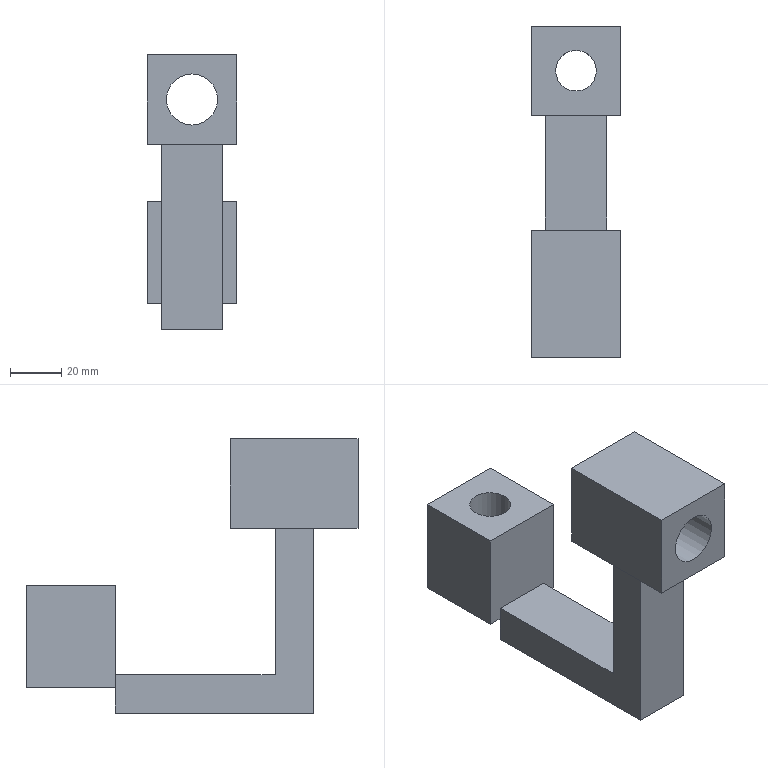Component | NX | 6 | 1 solid | 21 faces | volume 135136 mm3 | plane 19 | cylinder 2 | commonest cylinder face diameters 20 x1 16 x1